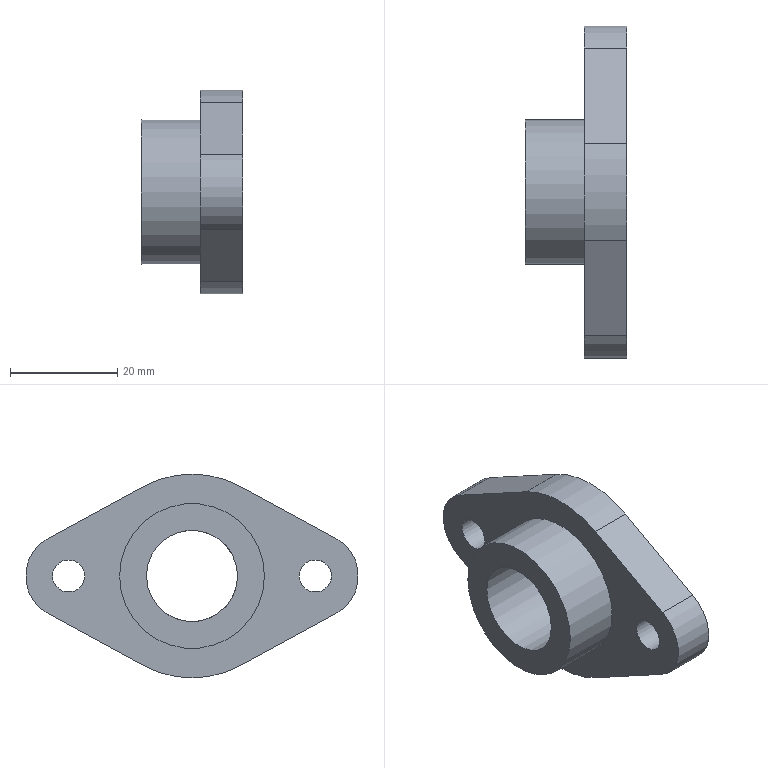Component | NX | OUTER_END_CAP | 1 solid | 15 faces | volume 14237 mm3 | cylinder 8 | plane 7 | commonest cylinder face diameters 16 x2 38 x2 6 x2 27 x1 17 x1